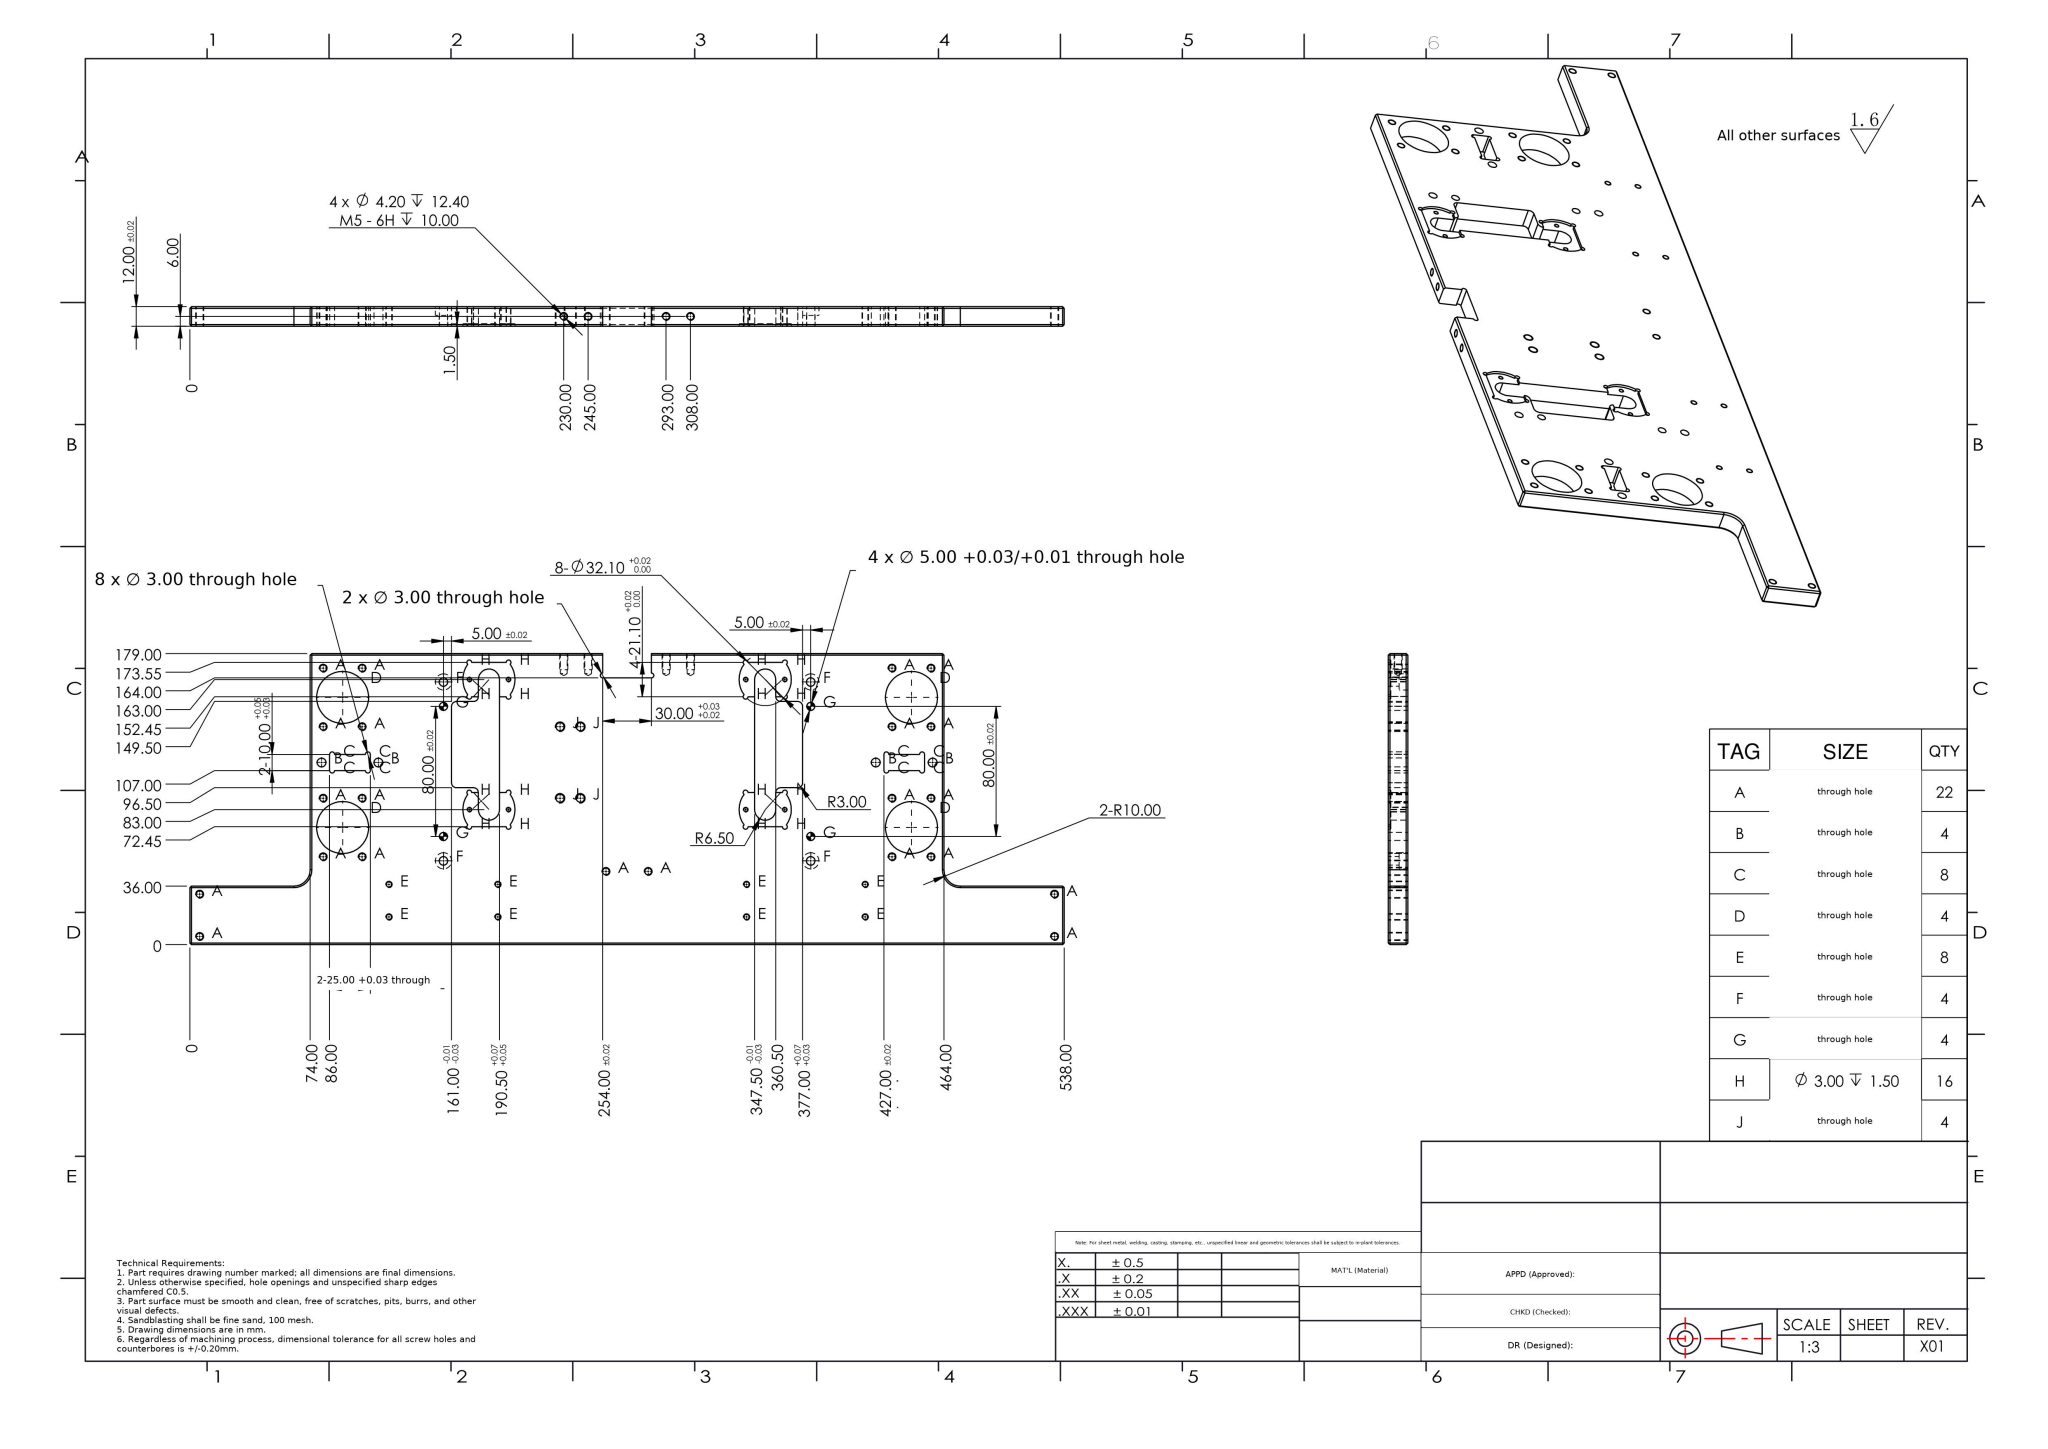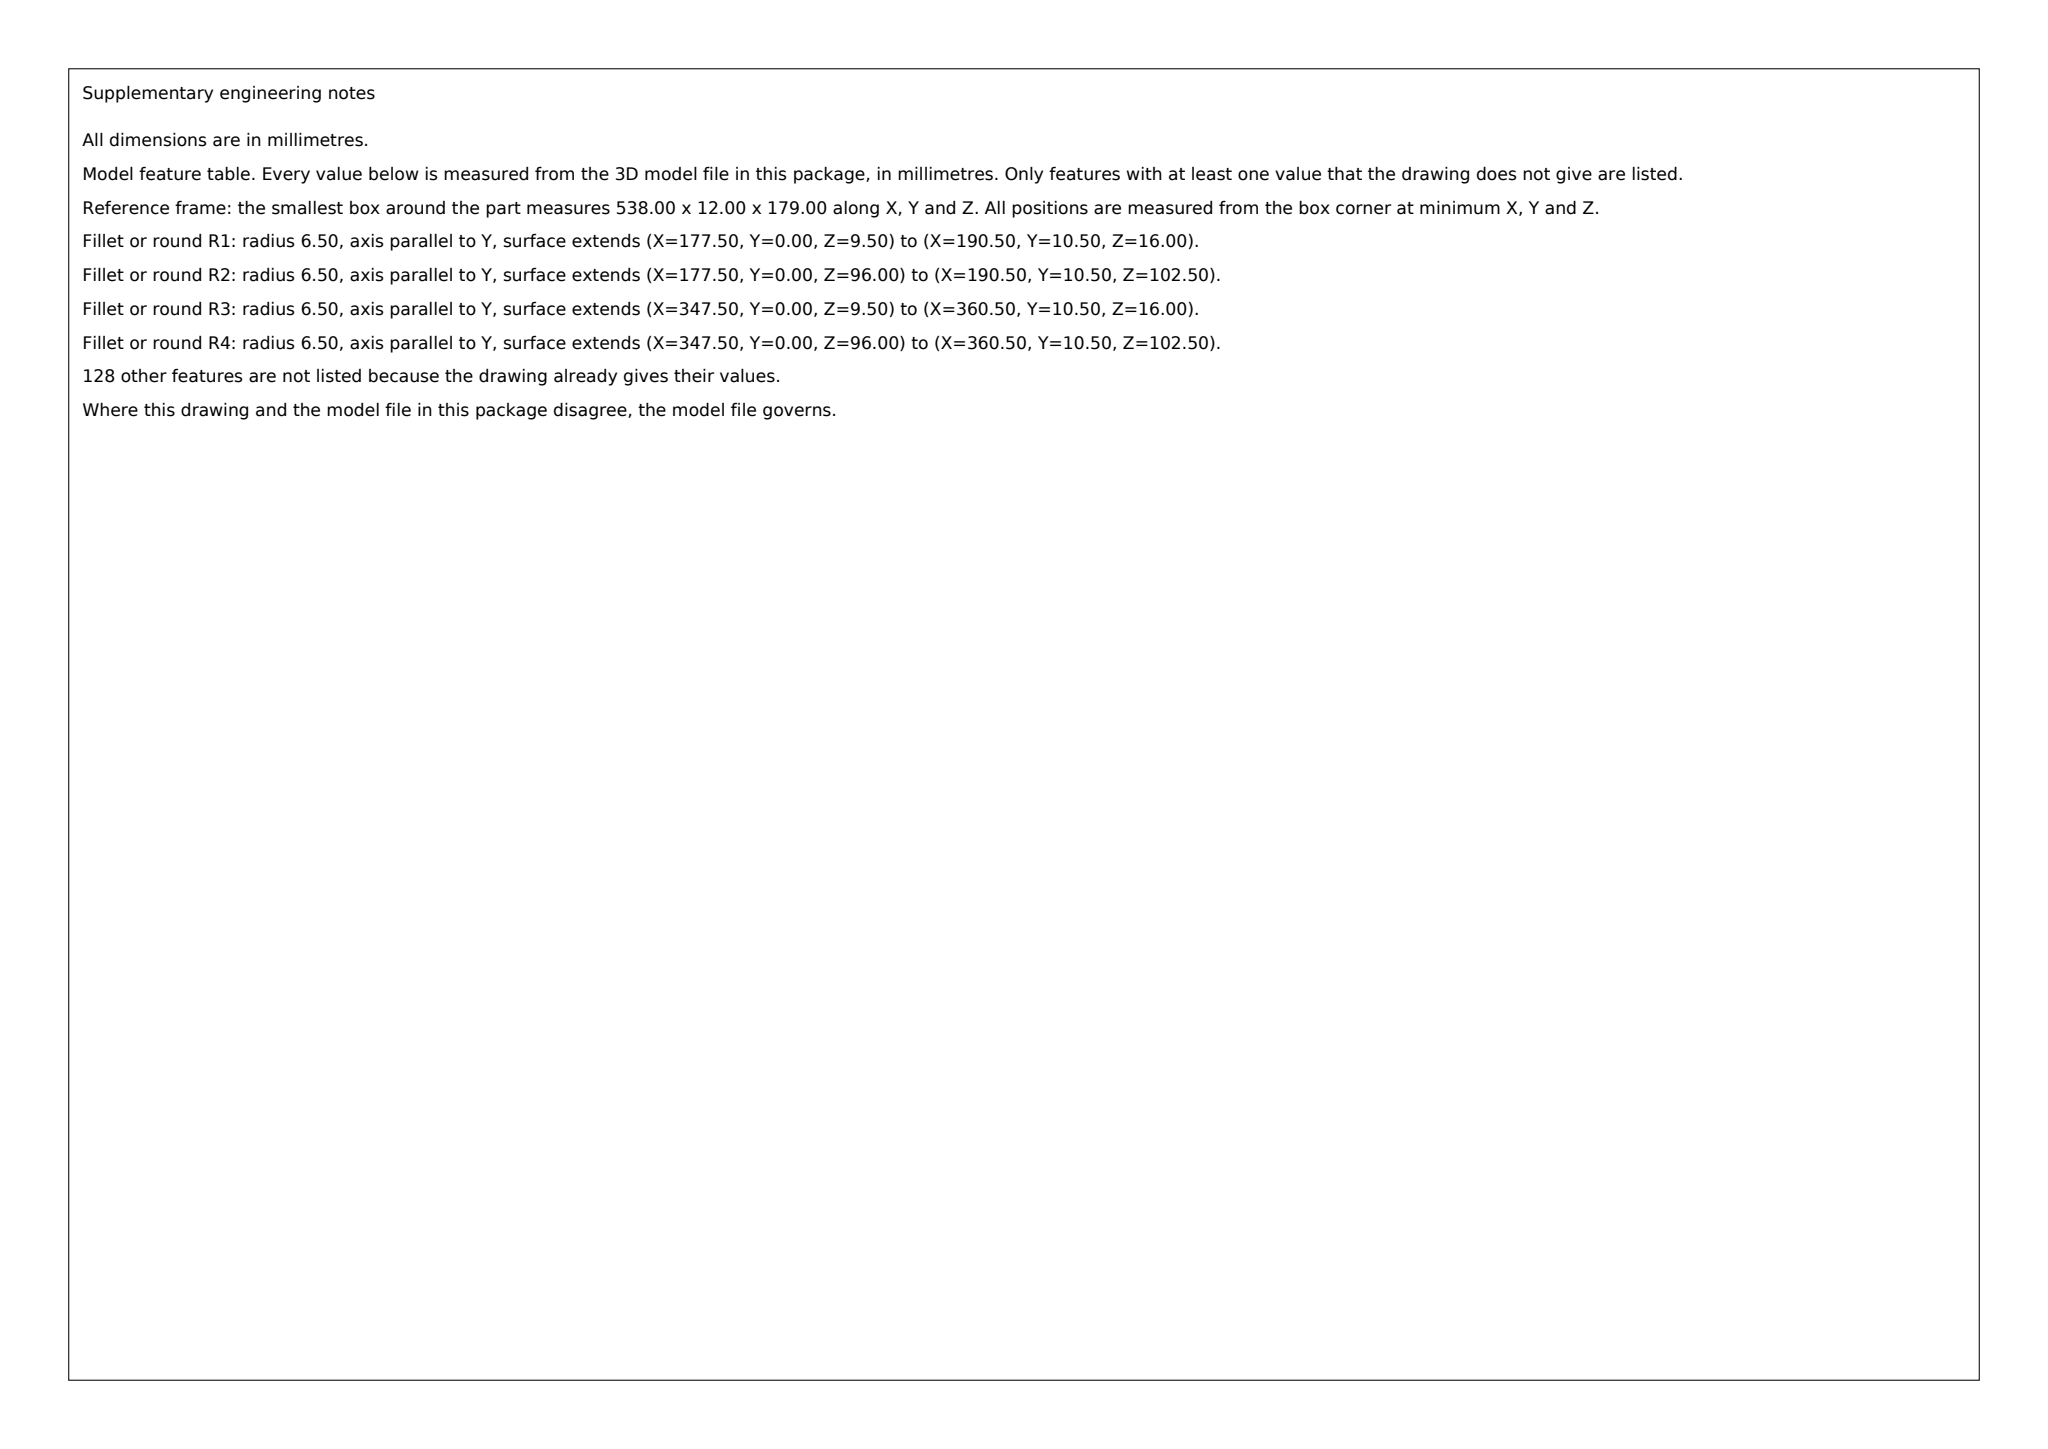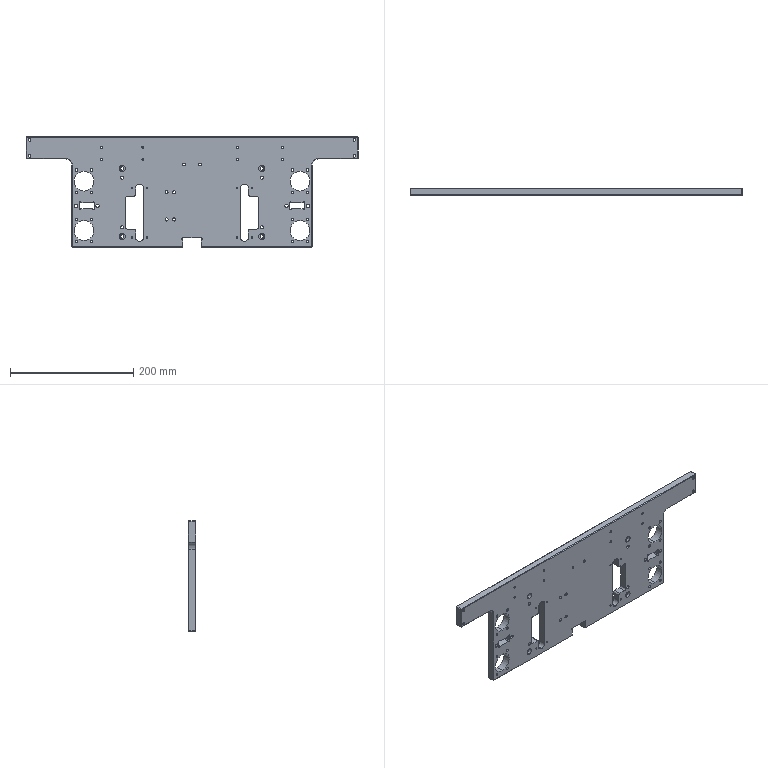Part | SolidWorks | mm | 1 solid | 296 faces | box 538 x 12 x 179 mm | volume 787643 mm3 | cylinder 194 | plane 90 | cone 12 | commonest cylinder face diameters 4.2 x52 3 x38 2.5 x16 3.3 x16 5 x16 5.5 x8 10 x8 5.3 x8